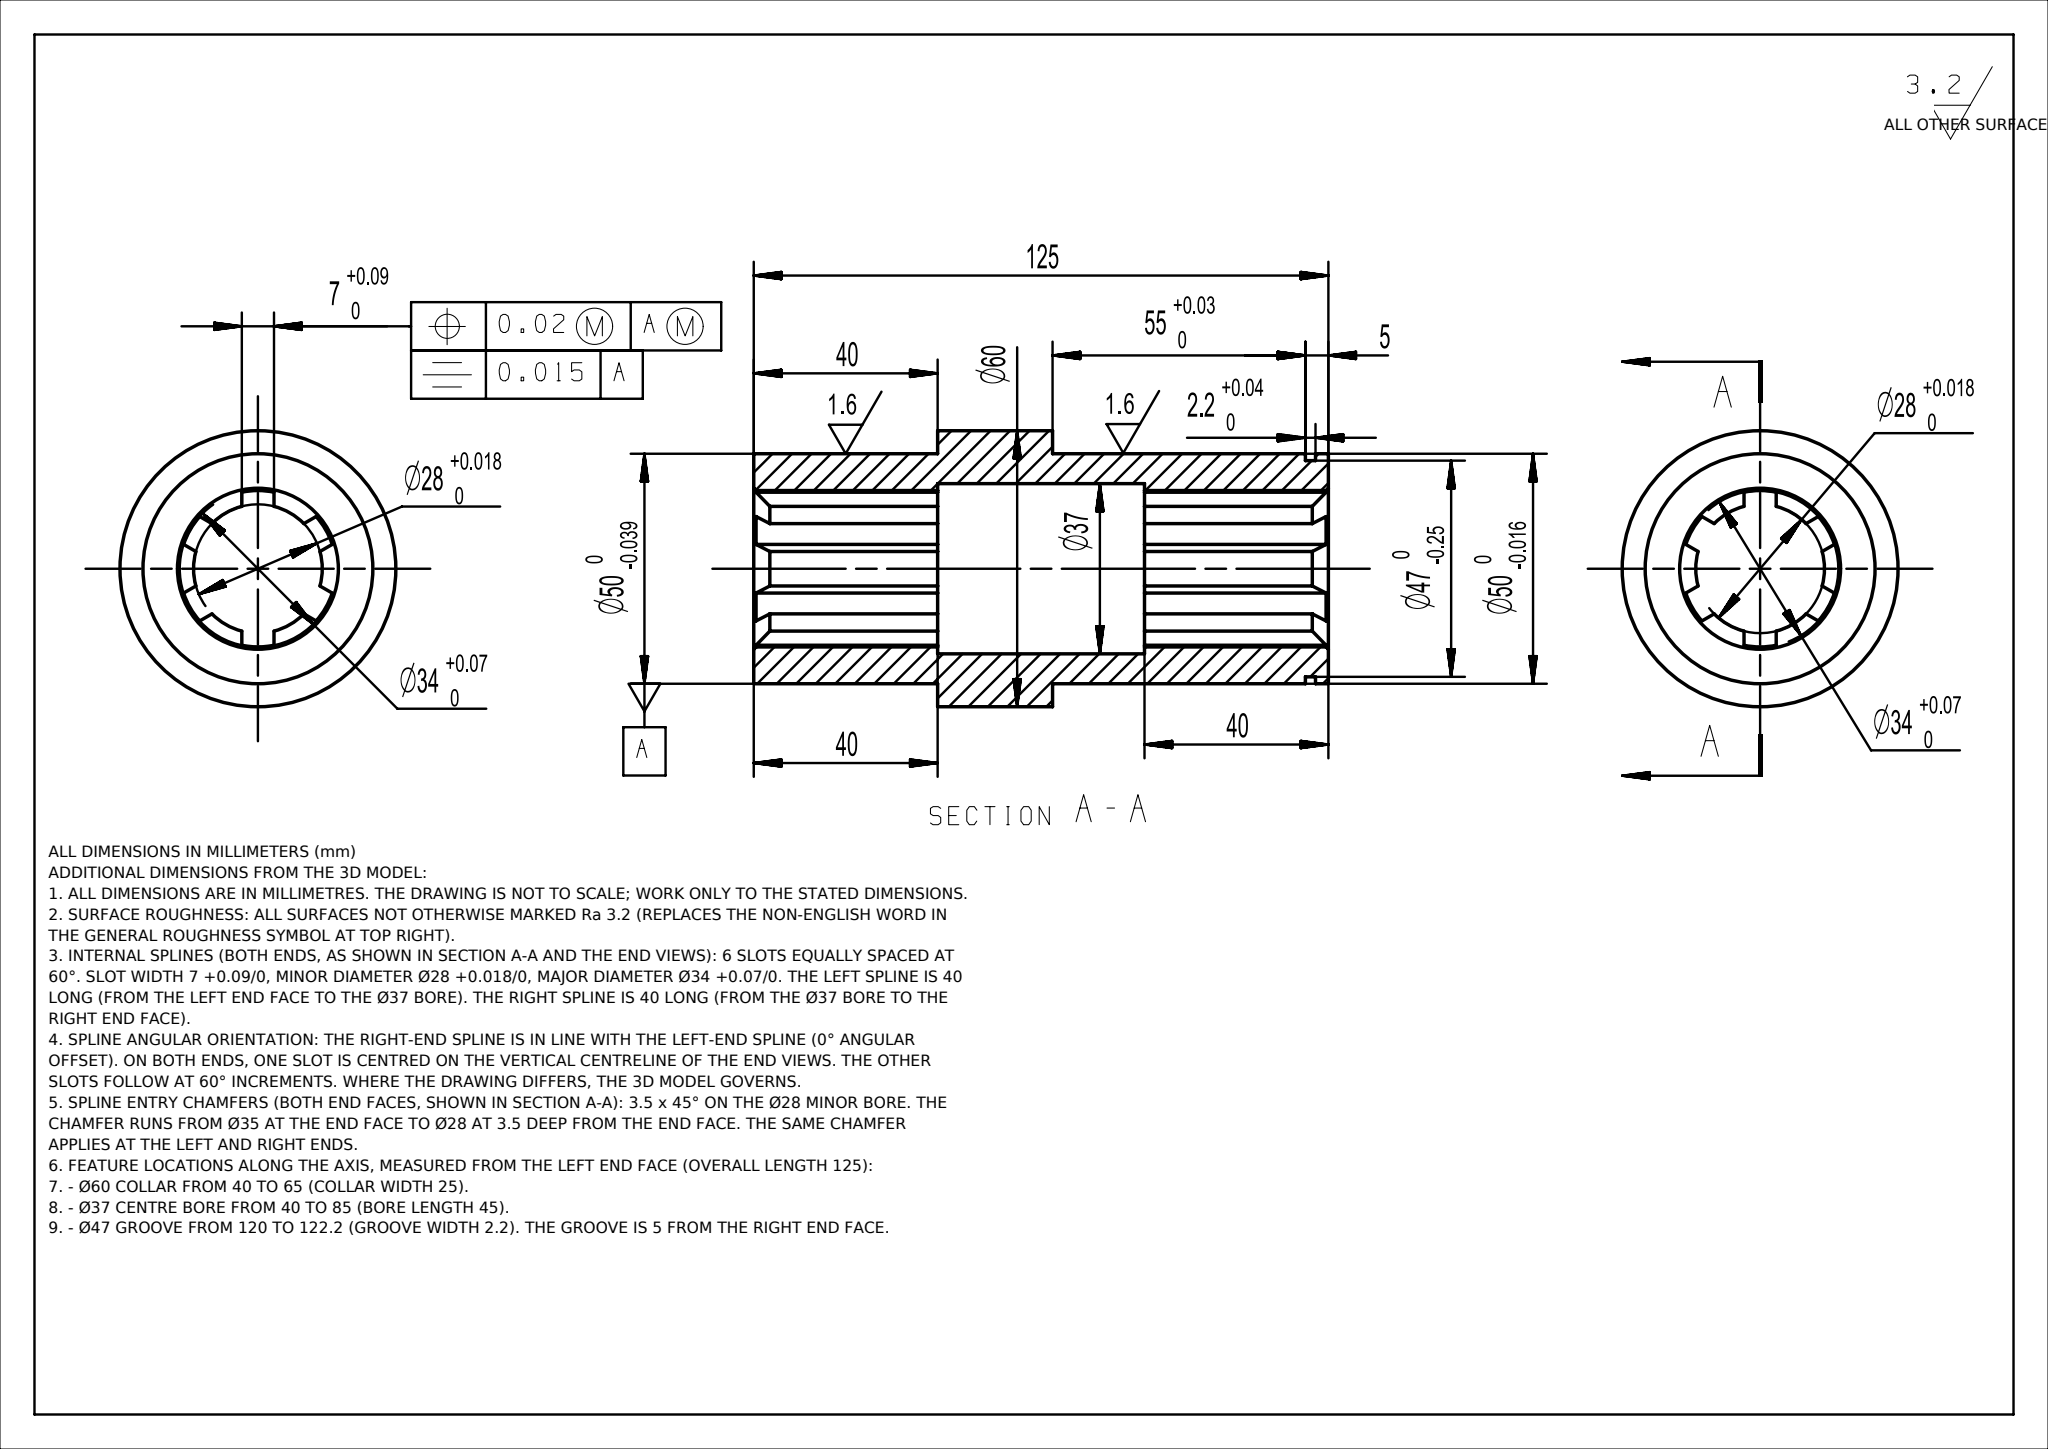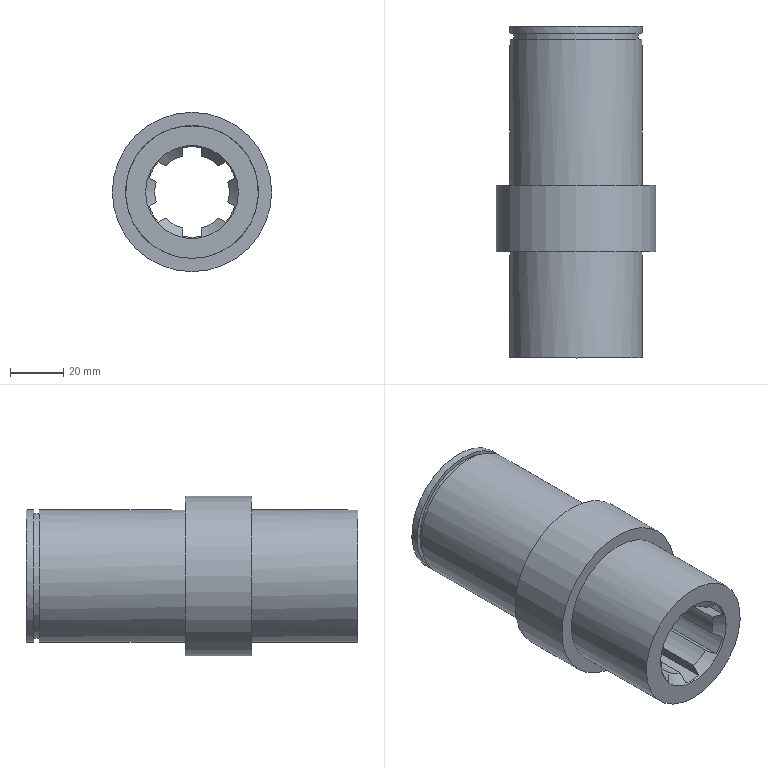Part | NX | mm | 1 solid | 64 faces | box 60 x 125 x 60 mm | volume 158036 mm3 | plane 32 | cylinder 30 | cone 2 | commonest cylinder face diameters 34 x12 28 x12 50 x3 60 x1 37 x1 47 x1